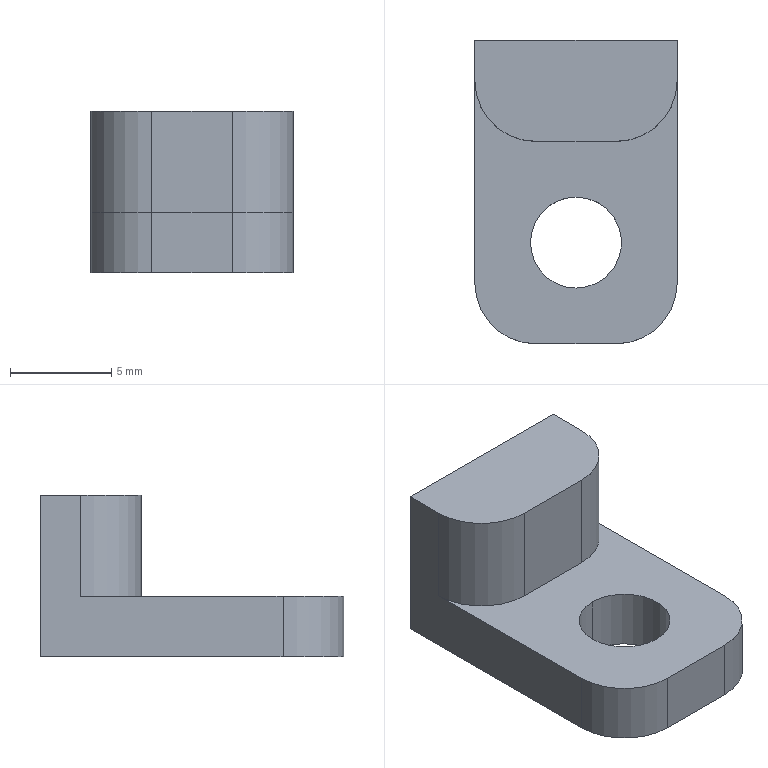CAM job | Mastercam | mm | 11 operations | part box 10 x 15 x 8
1. Facing | 10 - 10 平铣刀
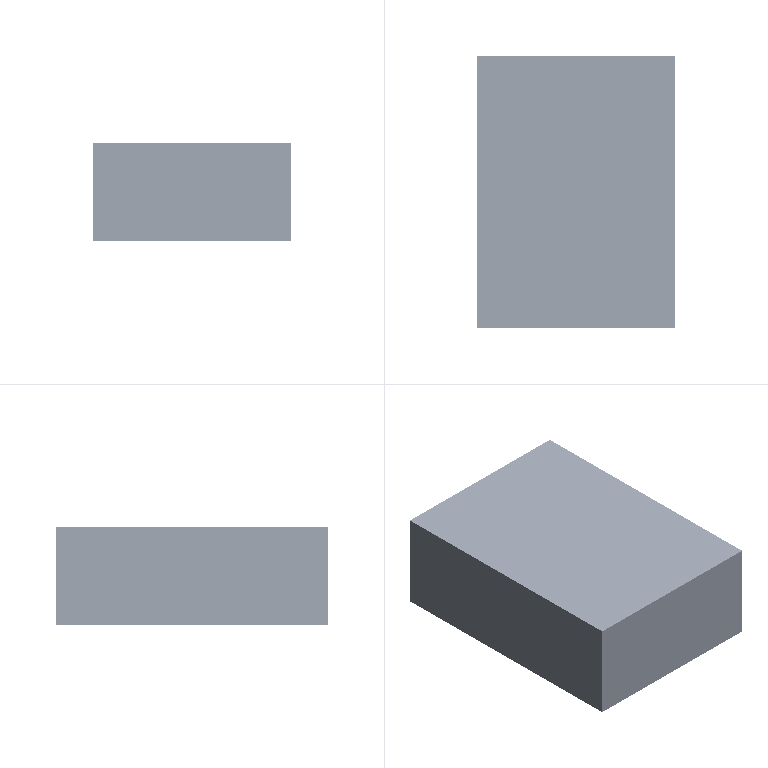2. Contour (Ramp) | 10 - 10 平铣刀
3. Contour (2D) | 10 - 10 平铣刀
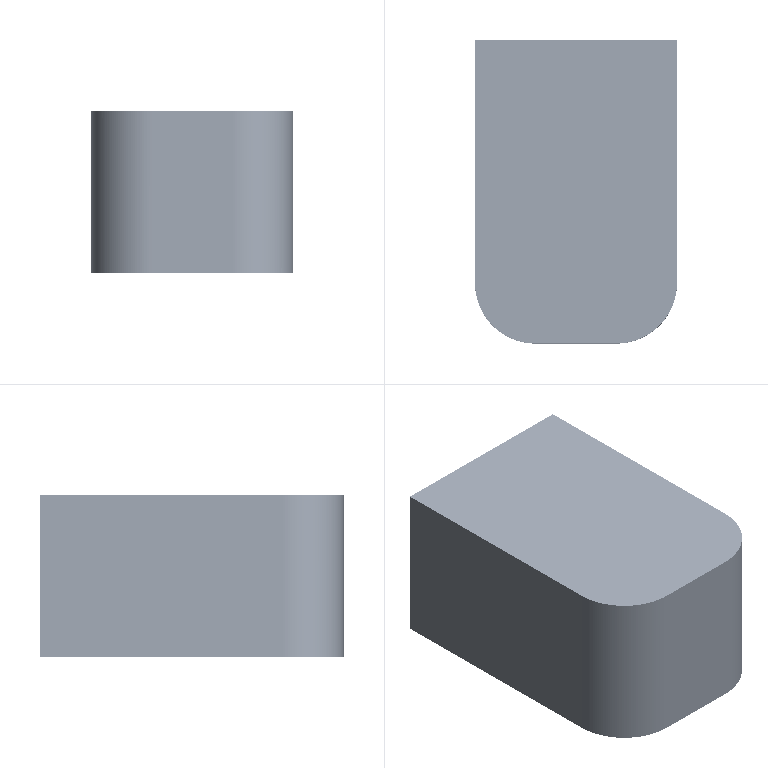4. Drill/Counterbore | 7 - 4 倒角刀
5. Contour (2D chamfer) | 7 - 4 倒角刀
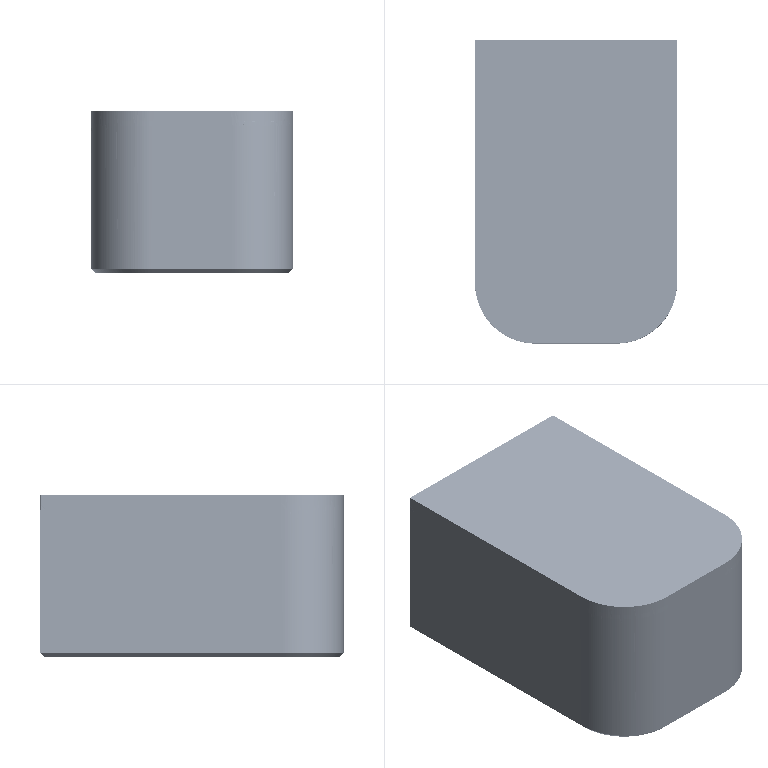6. Facing | 10 - 10 平铣刀
7. Contour (Ramp) | 10 - 10 平铣刀
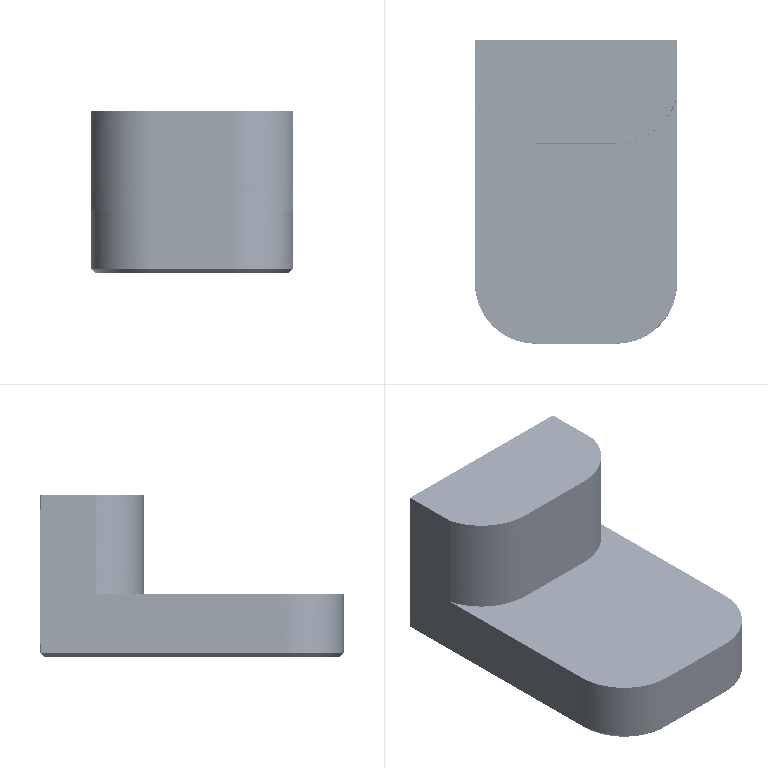8. Contour (2D) | 10 - 10 平铣刀
9. Drill/Counterbore | 7 - 4 倒角刀
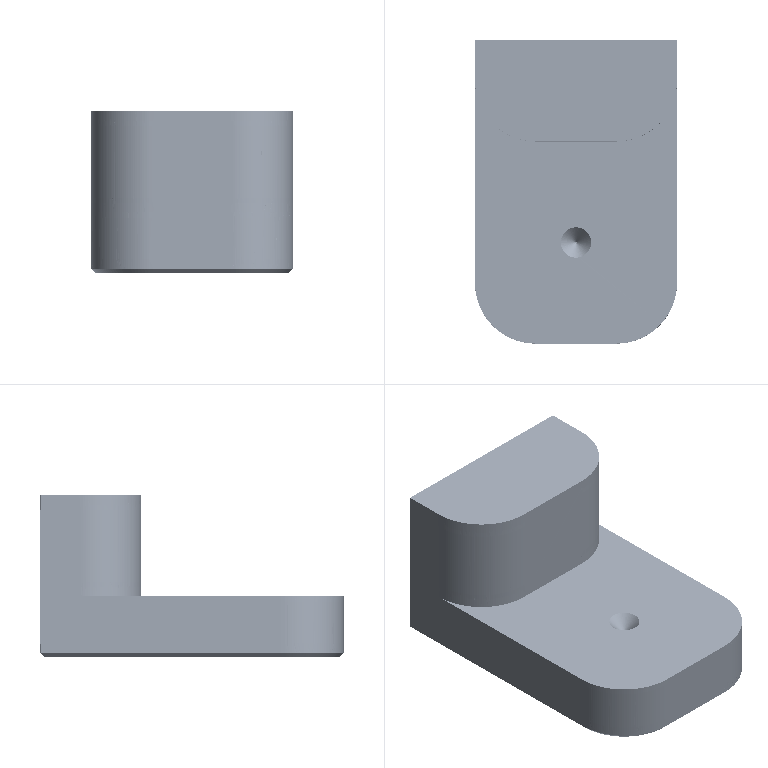10. Contour (2D chamfer) | 7 - 4 倒角刀
11. Drill/Counterbore | 7 - 4 倒角刀